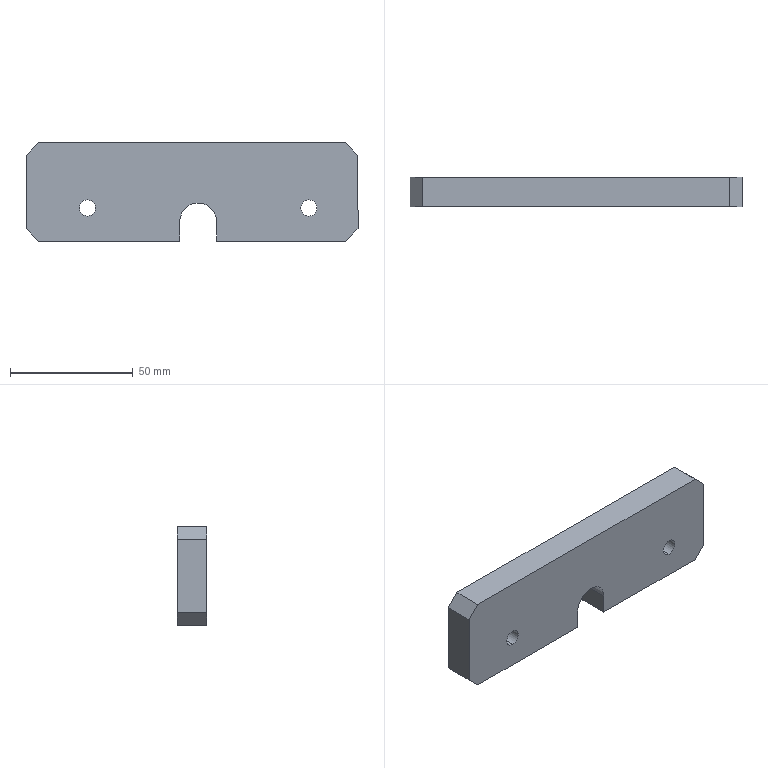Component | SolidWorks | PressingMechanism-26-1 | 1 solid | 18 faces | box 135 x 12 x 40 mm | volume 60879 mm3 | plane 13 | cylinder 5 | commonest cylinder face diameters 6.6 x4 15 x1
build123d program:
from build123d import *

# Parameters (mm, degrees)
SKETCH1_W               = 140
SKETCH1_H               = 50
EXTRUDE1_DEPTH          = 6
M6_CLEARANCE_HOLE1_D    = 6.6
CUT_EXTRUDE1_DEPTH      = 76.293
SKETCH2_W               = 140
SKETCH2_H               = 12.913
CUT_EXTRUDE1_2_DEPTH    = 25
CHAMFER1_SIZE           = 5
CUT_EXTRUDE2_DEPTH      = 76.293
CUT_EXTRUDE2_DEPTH_BACK = 76.293
CHAMFER1_2_SIZE         = 5


with BuildPart() as part:
    # Sketch1 → Extrude1 (new, symmetric)
    with BuildSketch(Plane(origin=(0, 0, 0), x_dir=(1, 0, 0), z_dir=(0, 1, 0))):
        Rectangle(SKETCH1_W, SKETCH1_H)
    extrude(amount=EXTRUDE1_DEPTH, both=True)

    # M6 Clearance Hole1 (through all)
    with Locations(Plane(origin=(0, -6, 0), x_dir=(-1, 0, 0), z_dir=(0, -1, 0))):
        with Locations((45, -1.5), (-45, -1.5)):
            Hole(M6_CLEARANCE_HOLE1_D / 2)

    # Sketch7 → Cut-Extrude1 (cut, through all)
    with BuildSketch(Plane(origin=(0, 6, 0), x_dir=(1, 0, 0), z_dir=(0, 1, 0))):
        with BuildLine():
            Line((7.5, -25), (7.5, -7))
            ThreePointArc((7.5, -7), (0, 0.5), (-7.5, -7))
            Line((-7.5, -7), (-7.5, -25))
            Line((-7.5, -25), (7.5, -25))
        make_face()
    extrude(amount=-CUT_EXTRUDE1_DEPTH, mode=Mode.SUBTRACT)

    # Sketch2 → Cut-Extrude1_2 (cut)
    with BuildSketch(Plane(origin=(0, 6, 0), x_dir=(1, 0, 0), z_dir=(0, 1, 0))):
        with Locations((0, -21.457)):
            Rectangle(SKETCH2_W, SKETCH2_H)
    extrude(amount=-CUT_EXTRUDE1_2_DEPTH, mode=Mode.SUBTRACT)

    # Chamfer1
    chamfer1_edges = [part.edges().sort_by_distance(p)[0] for p in [
        (70, 0, 15),
        (-70, 0, 15),
        (-70, 0, -25),
        (70, 0, -25),
    ]]
    chamfer(chamfer1_edges, length=CHAMFER1_SIZE)

    # Sketch3_2 → Cut-Extrude2 (cut, two sides: drawn at the far end of the back side and taken through both)
    with BuildSketch(Plane.XZ.offset(6).offset(-CUT_EXTRUDE2_DEPTH_BACK)):
        Polygon((65, 307.002), (65, 15), (65, -25.698), (65, -317.7), (649.005, -317.7), (649.005, 307.002), align=None)
    extrude(amount=CUT_EXTRUDE2_DEPTH + CUT_EXTRUDE2_DEPTH_BACK, mode=Mode.SUBTRACT)

    # Chamfer1_2
    chamfer1_2_edges = [part.edges().sort_by_distance(p)[0] for p in [
        (65, 0, 15),
        (65, 0, -25),
    ]]
    chamfer(chamfer1_2_edges, length=CHAMFER1_2_SIZE)


solid = part.part

# Placed as in the assembly
solid = solid.moved(Location((45, -265, 62.5), (180, 0, 0)))
STEP:
#1=COLOUR_RGB('',0.7922,0.8196,0.9333);
#2=FILL_AREA_STYLE_COLOUR('',#1);
#3=FILL_AREA_STYLE('',(#2));
#4=SURFACE_STYLE_FILL_AREA(#3);
#5=SURFACE_SIDE_STYLE('',(#4));
#6=SURFACE_STYLE_USAGE(.BOTH.,#5);
#7=PRESENTATION_STYLE_ASSIGNMENT((#6));
#8=CARTESIAN_POINT('',(-0.,-10.669,2.272));
#9=VERTEX_POINT('',#8);
#10=CARTESIAN_POINT('',(-0.,-10.669,2.531));
#11=VERTEX_POINT('',#10);
#12=CARTESIAN_POINT('',(-0.,-10.669,2.402));
#13=DIRECTION('',(0.,1.,0.));
#14=DIRECTION('',(-0.,0.,1.));
#15=AXIS2_PLACEMENT_3D('',#12,#13,#14);
#16=CIRCLE('',#15,0.1299);
#17=EDGE_CURVE('',#9,#11,#16,.T.);
#18=ORIENTED_EDGE('',*,*,#17,.F.);
#19=CARTESIAN_POINT('',(-0.,-10.197,2.272));
#20=VERTEX_POINT('',#19);
#21=CARTESIAN_POINT('',(-0.,-10.197,2.272));
#22=DIRECTION('',(0.,1.,0.));
#23=VECTOR('',#22,39.37);
#24=LINE('',#21,#23);
#25=EDGE_CURVE('',#9,#20,#24,.T.);
#26=ORIENTED_EDGE('',*,*,#25,.T.);
#27=CARTESIAN_POINT('',(-0.,-10.197,2.531));
#28=VERTEX_POINT('',#27);
#29=CARTESIAN_POINT('',(-0.,-10.197,2.402));
#30=DIRECTION('',(0.,1.,0.));
#31=DIRECTION('',(-0.,0.,1.));
#32=AXIS2_PLACEMENT_3D('',#29,#30,#31);
#33=CIRCLE('',#32,0.1299);
#34=EDGE_CURVE('',#20,#28,#33,.T.);
#35=ORIENTED_EDGE('',*,*,#34,.T.);
#36=CARTESIAN_POINT('',(-0.,-10.197,2.531));
#37=DIRECTION('',(0.,1.,0.));
#38=VECTOR('',#37,39.37);
#39=LINE('',#36,#38);
#40=EDGE_CURVE('',#11,#28,#39,.T.);
#41=ORIENTED_EDGE('',*,*,#40,.F.);
#42=EDGE_LOOP('',(#18,#26,#35,#41));
#43=FACE_OUTER_BOUND('',#42,.T.);
#44=CARTESIAN_POINT('',(-0.,-10.197,2.402));
#45=DIRECTION('',(0.,1.,0.));
#46=DIRECTION('',(-0.,0.,1.));
#47=AXIS2_PLACEMENT_3D('',#44,#45,#46);
#48=CYLINDRICAL_SURFACE('',#47,0.1299);
#49=ADVANCED_FACE('',(#43),#48,.F.);
#50=CARTESIAN_POINT('',(3.543,-10.669,2.272));
#51=VERTEX_POINT('',#50);
#52=CARTESIAN_POINT('',(3.543,-10.669,2.531));
#53=VERTEX_POINT('',#52);
#54=CARTESIAN_POINT('',(3.543,-10.669,2.402));
#55=DIRECTION('',(0.,1.,0.));
#56=DIRECTION('',(0.,0.,1.));
#57=AXIS2_PLACEMENT_3D('',#54,#55,#56);
#58=CIRCLE('',#57,0.1299);
#59=EDGE_CURVE('',#51,#53,#58,.T.);
#60=ORIENTED_EDGE('',*,*,#59,.F.);
#61=CARTESIAN_POINT('',(3.543,-10.197,2.272));
#62=VERTEX_POINT('',#61);
#63=CARTESIAN_POINT('',(3.543,-10.197,2.272));
#64=DIRECTION('',(0.,1.,0.));
#65=VECTOR('',#64,39.37);
#66=LINE('',#63,#65);
#67=EDGE_CURVE('',#51,#62,#66,.T.);
#68=ORIENTED_EDGE('',*,*,#67,.T.);
#69=CARTESIAN_POINT('',(3.543,-10.197,2.531));
#70=VERTEX_POINT('',#69);
#71=CARTESIAN_POINT('',(3.543,-10.197,2.402));
#72=DIRECTION('',(0.,1.,0.));
#73=DIRECTION('',(0.,0.,1.));
#74=AXIS2_PLACEMENT_3D('',#71,#72,#73);
#75=CIRCLE('',#74,0.1299);
#76=EDGE_CURVE('',#62,#70,#75,.T.);
#77=ORIENTED_EDGE('',*,*,#76,.T.);
#78=CARTESIAN_POINT('',(3.543,-10.197,2.531));
#79=DIRECTION('',(0.,1.,0.));
#80=VECTOR('',#79,39.37);
#81=LINE('',#78,#80);
#82=EDGE_CURVE('',#53,#70,#81,.T.);
#83=ORIENTED_EDGE('',*,*,#82,.F.);
#84=EDGE_LOOP('',(#60,#68,#77,#83));
#85=FACE_OUTER_BOUND('',#84,.T.);
#86=CARTESIAN_POINT('',(3.543,-10.197,2.402));
#87=DIRECTION('',(0.,1.,0.));
#88=DIRECTION('',(0.,0.,1.));
#89=AXIS2_PLACEMENT_3D('',#86,#87,#88);
#90=CYLINDRICAL_SURFACE('',#89,0.1299);
#91=ADVANCED_FACE('',(#85),#90,.F.);
#92=CARTESIAN_POINT('',(-0.,-10.669,2.402));
#93=DIRECTION('',(0.,1.,0.));
#94=DIRECTION('',(-0.,0.,1.));
#95=AXIS2_PLACEMENT_3D('',#92,#93,#94);
#96=CIRCLE('',#95,0.1299);
#97=EDGE_CURVE('',#11,#9,#96,.T.);
#98=ORIENTED_EDGE('',*,*,#97,.T.);
#99=ORIENTED_EDGE('',*,*,#17,.T.);
#100=EDGE_LOOP('',(#98,#99));
#101=FACE_BOUND('',#100,.T.);
#102=CARTESIAN_POINT('',(3.543,-10.669,2.402));
#103=DIRECTION('',(0.,1.,0.));
#104=DIRECTION('',(0.,0.,1.));
#105=AXIS2_PLACEMENT_3D('',#102,#103,#104);
#106=CIRCLE('',#105,0.1299);
#107=EDGE_CURVE('',#53,#51,#106,.T.);
#108=ORIENTED_EDGE('',*,*,#107,.T.);
#109=ORIENTED_EDGE('',*,*,#59,.T.);
#110=EDGE_LOOP('',(#108,#109));
#111=FACE_BOUND('',#110,.T.);
#112=CARTESIAN_POINT('',(4.331,-10.669,2.067));
#113=VERTEX_POINT('',#112);
#114=CARTESIAN_POINT('',(4.331,-10.669,3.248));
#115=VERTEX_POINT('',#114);
#116=CARTESIAN_POINT('',(4.331,-10.669,2.461));
#117=DIRECTION('',(-0.,-0.,1.));
#118=VECTOR('',#117,39.37);
#119=LINE('',#116,#118);
#120=EDGE_CURVE('',#113,#115,#119,.T.);
#121=ORIENTED_EDGE('',*,*,#120,.T.);
#122=CARTESIAN_POINT('',(4.134,-10.669,3.445));
#123=VERTEX_POINT('',#122);
#124=CARTESIAN_POINT('',(3.445,-10.669,4.134));
#125=DIRECTION('',(-0.7071,-0.,0.7071));
#126=VECTOR('',#125,39.37);
#127=LINE('',#124,#126);
#128=EDGE_CURVE('',#115,#123,#127,.T.);
#129=ORIENTED_EDGE('',*,*,#128,.T.);
#130=CARTESIAN_POINT('',(-0.7874,-10.669,3.445));
#131=VERTEX_POINT('',#130);
#132=CARTESIAN_POINT('',(-0.9843,-10.669,3.445));
#133=DIRECTION('',(-1.,0.,-0.));
#134=VECTOR('',#133,39.37);
#135=LINE('',#132,#134);
#136=EDGE_CURVE('',#123,#131,#135,.T.);
#137=ORIENTED_EDGE('',*,*,#136,.T.);
#138=CARTESIAN_POINT('',(-0.9843,-10.669,3.248));
#139=VERTEX_POINT('',#138);
#140=CARTESIAN_POINT('',(0.,-10.669,4.232));
#141=DIRECTION('',(-0.7071,0.,-0.7071));
#142=VECTOR('',#141,39.37);
#143=LINE('',#140,#142);
#144=EDGE_CURVE('',#131,#139,#143,.T.);
#145=ORIENTED_EDGE('',*,*,#144,.T.);
#146=CARTESIAN_POINT('',(-0.9843,-10.669,2.067));
#147=VERTEX_POINT('',#146);
#148=CARTESIAN_POINT('',(-0.9843,-10.669,3.445));
#149=DIRECTION('',(0.,0.,-1.));
#150=VECTOR('',#149,39.37);
#151=LINE('',#148,#150);
#152=EDGE_CURVE('',#139,#147,#151,.T.);
#153=ORIENTED_EDGE('',*,*,#152,.T.);
#154=CARTESIAN_POINT('',(-0.7874,-10.669,1.87));
#155=VERTEX_POINT('',#154);
#156=CARTESIAN_POINT('',(0.1969,-10.669,0.8858));
#157=DIRECTION('',(0.7071,0.,-0.7071));
#158=VECTOR('',#157,39.37);
#159=LINE('',#156,#158);
#160=EDGE_CURVE('',#147,#155,#159,.T.);
#161=ORIENTED_EDGE('',*,*,#160,.T.);
#162=CARTESIAN_POINT('',(1.476,-10.669,1.87));
#163=VERTEX_POINT('',#162);
#164=CARTESIAN_POINT('',(-0.9843,-10.669,1.87));
#165=DIRECTION('',(-1.,0.,-0.));
#166=VECTOR('',#165,39.37);
#167=LINE('',#164,#166);
#168=EDGE_CURVE('',#163,#155,#167,.T.);
#169=ORIENTED_EDGE('',*,*,#168,.F.);
#170=CARTESIAN_POINT('',(1.476,-10.669,2.185));
#171=VERTEX_POINT('',#170);
#172=CARTESIAN_POINT('',(1.476,-10.669,1.476));
#173=DIRECTION('',(-0.,0.,-1.));
#174=VECTOR('',#173,39.37);
#175=LINE('',#172,#174);
#176=EDGE_CURVE('',#171,#163,#175,.T.);
#177=ORIENTED_EDGE('',*,*,#176,.F.);
#178=CARTESIAN_POINT('',(2.067,-10.669,2.185));
#179=VERTEX_POINT('',#178);
#180=CARTESIAN_POINT('',(1.772,-10.669,2.185));
#181=DIRECTION('',(-0.,-1.,-0.));
#182=DIRECTION('',(0.,0.,1.));
#183=AXIS2_PLACEMENT_3D('',#180,#181,#182);
#184=CIRCLE('',#183,0.2953);
#185=EDGE_CURVE('',#179,#171,#184,.T.);
#186=ORIENTED_EDGE('',*,*,#185,.F.);
#187=CARTESIAN_POINT('',(2.067,-10.669,1.87));
#188=VERTEX_POINT('',#187);
#189=CARTESIAN_POINT('',(2.067,-10.669,1.476));
#190=DIRECTION('',(-0.,-0.,1.));
#191=VECTOR('',#190,39.37);
#192=LINE('',#189,#191);
#193=EDGE_CURVE('',#188,#179,#192,.T.);
#194=ORIENTED_EDGE('',*,*,#193,.F.);
#195=CARTESIAN_POINT('',(4.134,-10.669,1.87));
#196=VERTEX_POINT('',#195);
#197=CARTESIAN_POINT('',(-0.9843,-10.669,1.87));
#198=DIRECTION('',(-1.,0.,-0.));
#199=VECTOR('',#198,39.37);
#200=LINE('',#197,#199);
#201=EDGE_CURVE('',#196,#188,#200,.T.);
#202=ORIENTED_EDGE('',*,*,#201,.F.);
#203=CARTESIAN_POINT('',(3.248,-10.669,0.9843));
#204=DIRECTION('',(0.7071,-0.,0.7071));
#205=VECTOR('',#204,39.37);
#206=LINE('',#203,#205);
#207=EDGE_CURVE('',#196,#113,#206,.T.);
#208=ORIENTED_EDGE('',*,*,#207,.T.);
#209=EDGE_LOOP('',(#121,#129,#137,#145,#153,#161,#169,#177,#186,#194,#202,#208));
#210=FACE_OUTER_BOUND('',#209,.T.);
#211=CARTESIAN_POINT('',(1.772,-10.669,2.461));
#212=DIRECTION('',(-0.,-1.,-0.));
#213=DIRECTION('',(0.,0.,-1.));
#214=AXIS2_PLACEMENT_3D('',#211,#212,#213);
#215=PLANE('',#214);
#216=ADVANCED_FACE('',(#101,#111,#210),#215,.T.);
#217=CARTESIAN_POINT('',(3.543,-10.197,2.402));
#218=DIRECTION('',(0.,1.,0.));
#219=DIRECTION('',(0.,0.,1.));
#220=AXIS2_PLACEMENT_3D('',#217,#218,#219);
#221=CIRCLE('',#220,0.1299);
#222=EDGE_CURVE('',#70,#62,#221,.T.);
#223=ORIENTED_EDGE('',*,*,#222,.F.);
#224=ORIENTED_EDGE('',*,*,#76,.F.);
#225=EDGE_LOOP('',(#223,#224));
#226=FACE_BOUND('',#225,.T.);
#227=CARTESIAN_POINT('',(-0.,-10.197,2.402));
#228=DIRECTION('',(0.,1.,0.));
#229=DIRECTION('',(-0.,0.,1.));
#230=AXIS2_PLACEMENT_3D('',#227,#228,#229);
#231=CIRCLE('',#230,0.1299);
#232=EDGE_CURVE('',#28,#20,#231,.T.);
#233=ORIENTED_EDGE('',*,*,#232,.F.);
#234=ORIENTED_EDGE('',*,*,#34,.F.);
#235=EDGE_LOOP('',(#233,#234));
#236=FACE_BOUND('',#235,.T.);
#237=CARTESIAN_POINT('',(4.134,-10.197,3.445));
#238=VERTEX_POINT('',#237);
#239=CARTESIAN_POINT('',(-0.7874,-10.197,3.445));
#240=VERTEX_POINT('',#239);
#241=CARTESIAN_POINT('',(-0.9843,-10.197,3.445));
#242=DIRECTION('',(-1.,0.,-0.));
#243=VECTOR('',#242,39.37);
#244=LINE('',#241,#243);
#245=EDGE_CURVE('',#238,#240,#244,.T.);
#246=ORIENTED_EDGE('',*,*,#245,.F.);
#247=CARTESIAN_POINT('',(4.331,-10.197,3.248));
#248=VERTEX_POINT('',#247);
#249=CARTESIAN_POINT('',(4.134,-10.197,3.445));
#250=DIRECTION('',(0.7071,0.,-0.7071));
#251=VECTOR('',#250,39.37);
#252=LINE('',#249,#251);
#253=EDGE_CURVE('',#238,#248,#252,.T.);
#254=ORIENTED_EDGE('',*,*,#253,.T.);
#255=CARTESIAN_POINT('',(4.331,-10.197,2.067));
#256=VERTEX_POINT('',#255);
#257=CARTESIAN_POINT('',(4.331,-10.197,2.461));
#258=DIRECTION('',(-0.,-0.,1.));
#259=VECTOR('',#258,39.37);
#260=LINE('',#257,#259);
#261=EDGE_CURVE('',#256,#248,#260,.T.);
#262=ORIENTED_EDGE('',*,*,#261,.F.);
#263=CARTESIAN_POINT('',(4.134,-10.197,1.87));
#264=VERTEX_POINT('',#263);
#265=CARTESIAN_POINT('',(4.134,-10.197,1.87));
#266=DIRECTION('',(-0.7071,0.,-0.7071));
#267=VECTOR('',#266,39.37);
#268=LINE('',#265,#267);
#269=EDGE_CURVE('',#256,#264,#268,.T.);
#270=ORIENTED_EDGE('',*,*,#269,.T.);
#271=CARTESIAN_POINT('',(2.067,-10.197,1.87));
#272=VERTEX_POINT('',#271);
#273=CARTESIAN_POINT('',(1.772,-10.197,1.87));
#274=DIRECTION('',(-1.,0.,-0.));
#275=VECTOR('',#274,39.37);
#276=LINE('',#273,#275);
#277=EDGE_CURVE('',#264,#272,#276,.T.);
#278=ORIENTED_EDGE('',*,*,#277,.T.);
#279=CARTESIAN_POINT('',(2.067,-10.197,2.185));
#280=VERTEX_POINT('',#279);
#281=CARTESIAN_POINT('',(2.067,-10.197,1.476));
#282=DIRECTION('',(-0.,-0.,1.));
#283=VECTOR('',#282,39.37);
#284=LINE('',#281,#283);
#285=EDGE_CURVE('',#272,#280,#284,.T.);
#286=ORIENTED_EDGE('',*,*,#285,.T.);
#287=CARTESIAN_POINT('',(1.476,-10.197,2.185));
#288=VERTEX_POINT('',#287);
#289=CARTESIAN_POINT('',(1.772,-10.197,2.185));
#290=DIRECTION('',(-0.,-1.,-0.));
#291=DIRECTION('',(0.,0.,1.));
#292=AXIS2_PLACEMENT_3D('',#289,#290,#291);
#293=CIRCLE('',#292,0.2953);
#294=EDGE_CURVE('',#280,#288,#293,.T.);
#295=ORIENTED_EDGE('',*,*,#294,.T.);
#296=CARTESIAN_POINT('',(1.476,-10.197,1.87));
#297=VERTEX_POINT('',#296);
#298=CARTESIAN_POINT('',(1.476,-10.197,1.476));
#299=DIRECTION('',(-0.,0.,-1.));
#300=VECTOR('',#299,39.37);
#301=LINE('',#298,#300);
#302=EDGE_CURVE('',#288,#297,#301,.T.);
#303=ORIENTED_EDGE('',*,*,#302,.T.);
#304=CARTESIAN_POINT('',(-0.7874,-10.197,1.87));
#305=VERTEX_POINT('',#304);
#306=CARTESIAN_POINT('',(1.772,-10.197,1.87));
#307=DIRECTION('',(-1.,0.,-0.));
#308=VECTOR('',#307,39.37);
#309=LINE('',#306,#308);
#310=EDGE_CURVE('',#297,#305,#309,.T.);
#311=ORIENTED_EDGE('',*,*,#310,.T.);
#312=CARTESIAN_POINT('',(-0.9843,-10.197,2.067));
#313=VERTEX_POINT('',#312);
#314=CARTESIAN_POINT('',(-0.9843,-10.197,2.067));
#315=DIRECTION('',(-0.7071,-0.,0.7071));
#316=VECTOR('',#315,39.37);
#317=LINE('',#314,#316);
#318=EDGE_CURVE('',#305,#313,#317,.T.);
#319=ORIENTED_EDGE('',*,*,#318,.T.);
#320=CARTESIAN_POINT('',(-0.9843,-10.197,3.248));
#321=VERTEX_POINT('',#320);
#322=CARTESIAN_POINT('',(-0.9843,-10.197,3.445));
#323=DIRECTION('',(0.,0.,-1.));
#324=VECTOR('',#323,39.37);
#325=LINE('',#322,#324);
#326=EDGE_CURVE('',#321,#313,#325,.T.);
#327=ORIENTED_EDGE('',*,*,#326,.F.);
#328=CARTESIAN_POINT('',(-0.9843,-10.197,3.248));
#329=DIRECTION('',(0.7071,-0.,0.7071));
#330=VECTOR('',#329,39.37);
#331=LINE('',#328,#330);
#332=EDGE_CURVE('',#321,#240,#331,.T.);
#333=ORIENTED_EDGE('',*,*,#332,.T.);
#334=EDGE_LOOP('',(#246,#254,#262,#270,#278,#286,#295,#303,#311,#319,#327,#333));
#335=FACE_OUTER_BOUND('',#334,.T.);
#336=CARTESIAN_POINT('',(1.772,-10.197,2.461));
#337=DIRECTION('',(-0.,-1.,-0.));
#338=DIRECTION('',(0.,0.,-1.));
#339=AXIS2_PLACEMENT_3D('',#336,#337,#338);
#340=PLANE('',#339);
#341=ADVANCED_FACE('',(#226,#236,#335),#340,.F.);
#342=ORIENTED_EDGE('',*,*,#326,.T.);
#343=CARTESIAN_POINT('',(-0.9843,-10.669,2.067));
#344=DIRECTION('',(-0.,-1.,-0.));
#345=VECTOR('',#344,39.37);
#346=LINE('',#343,#345);
#347=EDGE_CURVE('',#313,#147,#346,.T.);
#348=ORIENTED_EDGE('',*,*,#347,.T.);
#349=ORIENTED_EDGE('',*,*,#152,.F.);
#350=CARTESIAN_POINT('',(-0.9843,-10.669,3.248));
#351=DIRECTION('',(0.,1.,0.));
#352=VECTOR('',#351,39.37);
#353=LINE('',#350,#352);
#354=EDGE_CURVE('',#139,#321,#353,.T.);
#355=ORIENTED_EDGE('',*,*,#354,.T.);
#356=EDGE_LOOP('',(#342,#348,#349,#355));
#357=FACE_OUTER_BOUND('',#356,.T.);
#358=CARTESIAN_POINT('',(-0.9843,-10.669,3.445));
#359=DIRECTION('',(1.,-0.,0.));
#360=DIRECTION('',(-0.,-0.,1.));
#361=AXIS2_PLACEMENT_3D('',#358,#359,#360);
#362=PLANE('',#361);
#363=ADVANCED_FACE('',(#357),#362,.F.);
#364=ORIENTED_EDGE('',*,*,#136,.F.);
#365=CARTESIAN_POINT('',(4.134,-10.197,3.445));
#366=DIRECTION('',(0.,1.,0.));
#367=VECTOR('',#366,39.37);
#368=LINE('',#365,#367);
#369=EDGE_CURVE('',#123,#238,#368,.T.);
#370=ORIENTED_EDGE('',*,*,#369,.T.);
#371=ORIENTED_EDGE('',*,*,#245,.T.);
#372=CARTESIAN_POINT('',(-0.7874,-10.669,3.445));
#373=DIRECTION('',(-0.,-1.,-0.));
#374=VECTOR('',#373,39.37);
#375=LINE('',#372,#374);
#376=EDGE_CURVE('',#240,#131,#375,.T.);
#377=ORIENTED_EDGE('',*,*,#376,.T.);
#378=EDGE_LOOP('',(#364,#370,#371,#377));
#379=FACE_OUTER_BOUND('',#378,.T.);
#380=CARTESIAN_POINT('',(-0.9843,-10.669,3.445));
#381=DIRECTION('',(0.,0.,-1.));
#382=DIRECTION('',(1.,-0.,0.));
#383=AXIS2_PLACEMENT_3D('',#380,#381,#382);
#384=PLANE('',#383);
#385=ADVANCED_FACE('',(#379),#384,.F.);
#386=ORIENTED_EDGE('',*,*,#67,.F.);
#387=ORIENTED_EDGE('',*,*,#107,.F.);
#388=ORIENTED_EDGE('',*,*,#82,.T.);
#389=ORIENTED_EDGE('',*,*,#222,.T.);
#390=EDGE_LOOP('',(#386,#387,#388,#389));
#391=FACE_OUTER_BOUND('',#390,.T.);
#392=CARTESIAN_POINT('',(3.543,-10.197,2.402));
#393=DIRECTION('',(0.,1.,0.));
#394=DIRECTION('',(0.,0.,1.));
#395=AXIS2_PLACEMENT_3D('',#392,#393,#394);
#396=CYLINDRICAL_SURFACE('',#395,0.1299);
#397=ADVANCED_FACE('',(#391),#396,.F.);
#398=ORIENTED_EDGE('',*,*,#25,.F.);
#399=ORIENTED_EDGE('',*,*,#97,.F.);
#400=ORIENTED_EDGE('',*,*,#40,.T.);
#401=ORIENTED_EDGE('',*,*,#232,.T.);
#402=EDGE_LOOP('',(#398,#399,#400,#401));
#403=FACE_OUTER_BOUND('',#402,.T.);
#404=CARTESIAN_POINT('',(-0.,-10.197,2.402));
#405=DIRECTION('',(0.,1.,0.));
#406=DIRECTION('',(-0.,0.,1.));
#407=AXIS2_PLACEMENT_3D('',#404,#405,#406);
#408=CYLINDRICAL_SURFACE('',#407,0.1299);
#409=ADVANCED_FACE('',(#403),#408,.F.);
#410=ORIENTED_EDGE('',*,*,#185,.T.);
#411=CARTESIAN_POINT('',(1.476,-10.197,2.185));
#412=DIRECTION('',(-0.,-1.,-0.));
#413=VECTOR('',#412,39.37);
#414=LINE('',#411,#413);
#415=EDGE_CURVE('',#288,#171,#414,.T.);
#416=ORIENTED_EDGE('',*,*,#415,.F.);
#417=ORIENTED_EDGE('',*,*,#294,.F.);
#418=CARTESIAN_POINT('',(2.067,-10.197,2.185));
#419=DIRECTION('',(-0.,-1.,-0.));
#420=VECTOR('',#419,39.37);
#421=LINE('',#418,#420);
#422=EDGE_CURVE('',#280,#179,#421,.T.);
#423=ORIENTED_EDGE('',*,*,#422,.T.);
#424=EDGE_LOOP('',(#410,#416,#417,#423));
#425=FACE_OUTER_BOUND('',#424,.T.);
#426=CARTESIAN_POINT('',(1.772,-10.197,2.185));
#427=DIRECTION('',(-0.,-1.,-0.));
#428=DIRECTION('',(0.,0.,-1.));
#429=AXIS2_PLACEMENT_3D('',#426,#427,#428);
#430=CYLINDRICAL_SURFACE('',#429,0.2953);
#431=ADVANCED_FACE('',(#425),#430,.F.);
#432=ORIENTED_EDGE('',*,*,#285,.F.);
#433=CARTESIAN_POINT('',(2.067,-10.197,1.87));
#434=DIRECTION('',(-0.,-1.,-0.));
#435=VECTOR('',#434,39.37);
#436=LINE('',#433,#435);
#437=EDGE_CURVE('',#272,#188,#436,.T.);
#438=ORIENTED_EDGE('',*,*,#437,.T.);
#439=ORIENTED_EDGE('',*,*,#193,.T.);
#440=ORIENTED_EDGE('',*,*,#422,.F.);
#441=EDGE_LOOP('',(#432,#438,#439,#440));
#442=FACE_OUTER_BOUND('',#441,.T.);
#443=CARTESIAN_POINT('',(2.067,-10.197,1.476));
#444=DIRECTION('',(1.,-0.,0.));
#445=DIRECTION('',(-0.,-0.,1.));
#446=AXIS2_PLACEMENT_3D('',#443,#444,#445);
#447=PLANE('',#446);
#448=ADVANCED_FACE('',(#442),#447,.F.);
#449=ORIENTED_EDGE('',*,*,#176,.T.);
#450=CARTESIAN_POINT('',(1.476,-10.197,1.87));
#451=DIRECTION('',(0.,1.,0.));
#452=VECTOR('',#451,39.37);
#453=LINE('',#450,#452);
#454=EDGE_CURVE('',#163,#297,#453,.T.);
#455=ORIENTED_EDGE('',*,*,#454,.T.);
#456=ORIENTED_EDGE('',*,*,#302,.F.);
#457=ORIENTED_EDGE('',*,*,#415,.T.);
#458=EDGE_LOOP('',(#449,#455,#456,#457));
#459=FACE_OUTER_BOUND('',#458,.T.);
#460=CARTESIAN_POINT('',(1.476,-10.197,1.476));
#461=DIRECTION('',(-1.,0.,0.));
#462=DIRECTION('',(-0.,0.,-1.));
#463=AXIS2_PLACEMENT_3D('',#460,#461,#462);
#464=PLANE('',#463);
#465=ADVANCED_FACE('',(#459),#464,.F.);
#466=ORIENTED_EDGE('',*,*,#168,.T.);
#467=CARTESIAN_POINT('',(-0.7874,-9.685,1.87));
#468=DIRECTION('',(0.,1.,0.));
#469=VECTOR('',#468,39.37);
#470=LINE('',#467,#469);
#471=EDGE_CURVE('',#155,#305,#470,.T.);
#472=ORIENTED_EDGE('',*,*,#471,.T.);
#473=ORIENTED_EDGE('',*,*,#310,.F.);
#474=ORIENTED_EDGE('',*,*,#454,.F.);
#475=EDGE_LOOP('',(#466,#472,#473,#474));
#476=FACE_OUTER_BOUND('',#475,.T.);
#477=CARTESIAN_POINT('',(-0.9843,-9.685,1.87));
#478=DIRECTION('',(-0.,-0.,1.));
#479=DIRECTION('',(-1.,0.,-0.));
#480=AXIS2_PLACEMENT_3D('',#477,#478,#479);
#481=PLANE('',#480);
#482=ADVANCED_FACE('',(#476),#481,.F.);
#483=ORIENTED_EDGE('',*,*,#277,.F.);
#484=CARTESIAN_POINT('',(4.134,-10.669,1.87));
#485=DIRECTION('',(-0.,-1.,-0.));
#486=VECTOR('',#485,39.37);
#487=LINE('',#484,#486);
#488=EDGE_CURVE('',#264,#196,#487,.T.);
#489=ORIENTED_EDGE('',*,*,#488,.T.);
#490=ORIENTED_EDGE('',*,*,#201,.T.);
#491=ORIENTED_EDGE('',*,*,#437,.F.);
#492=EDGE_LOOP('',(#483,#489,#490,#491));
#493=FACE_OUTER_BOUND('',#492,.T.);
#494=CARTESIAN_POINT('',(-0.9843,-9.685,1.87));
#495=DIRECTION('',(-0.,-0.,1.));
#496=DIRECTION('',(-1.,0.,-0.));
#497=AXIS2_PLACEMENT_3D('',#494,#495,#496);
#498=PLANE('',#497);
#499=ADVANCED_FACE('',(#493),#498,.F.);
#500=ORIENTED_EDGE('',*,*,#318,.F.);
#501=ORIENTED_EDGE('',*,*,#471,.F.);
#502=ORIENTED_EDGE('',*,*,#160,.F.);
#503=ORIENTED_EDGE('',*,*,#347,.F.);
#504=EDGE_LOOP('',(#500,#501,#502,#503));
#505=FACE_OUTER_BOUND('',#504,.T.);
#506=CARTESIAN_POINT('',(-0.9843,-10.669,2.067));
#507=DIRECTION('',(0.7071,-0.,0.7071));
#508=DIRECTION('',(-0.,-1.,-0.));
#509=AXIS2_PLACEMENT_3D('',#506,#507,#508);
#510=PLANE('',#509);
#511=ADVANCED_FACE('',(#505),#510,.F.);
#512=ORIENTED_EDGE('',*,*,#144,.F.);
#513=ORIENTED_EDGE('',*,*,#376,.F.);
#514=ORIENTED_EDGE('',*,*,#332,.F.);
#515=ORIENTED_EDGE('',*,*,#354,.F.);
#516=EDGE_LOOP('',(#512,#513,#514,#515));
#517=FACE_OUTER_BOUND('',#516,.T.);
#518=CARTESIAN_POINT('',(-0.9843,-10.669,3.248));
#519=DIRECTION('',(0.7071,0.,-0.7071));
#520=DIRECTION('',(0.,1.,0.));
#521=AXIS2_PLACEMENT_3D('',#518,#519,#520);
#522=PLANE('',#521);
#523=ADVANCED_FACE('',(#517),#522,.F.);
#524=ORIENTED_EDGE('',*,*,#261,.T.);
#525=CARTESIAN_POINT('',(4.331,-10.669,3.248));
#526=DIRECTION('',(-0.,-1.,-0.));
#527=VECTOR('',#526,39.37);
#528=LINE('',#525,#527);
#529=EDGE_CURVE('',#248,#115,#528,.T.);
#530=ORIENTED_EDGE('',*,*,#529,.T.);
#531=ORIENTED_EDGE('',*,*,#120,.F.);
#532=CARTESIAN_POINT('',(4.331,-10.197,2.067));
#533=DIRECTION('',(0.,1.,0.));
#534=VECTOR('',#533,39.37);
#535=LINE('',#532,#534);
#536=EDGE_CURVE('',#113,#256,#535,.T.);
#537=ORIENTED_EDGE('',*,*,#536,.T.);
#538=EDGE_LOOP('',(#524,#530,#531,#537));
#539=FACE_OUTER_BOUND('',#538,.T.);
#540=CARTESIAN_POINT('',(4.331,-3.007,1.87));
#541=DIRECTION('',(1.,-0.,0.));
#542=DIRECTION('',(-0.,-0.,1.));
#543=AXIS2_PLACEMENT_3D('',#540,#541,#542);
#544=PLANE('',#543);
#545=ADVANCED_FACE('',(#539),#544,.T.);
#546=ORIENTED_EDGE('',*,*,#128,.F.);
#547=ORIENTED_EDGE('',*,*,#529,.F.);
#548=ORIENTED_EDGE('',*,*,#253,.F.);
#549=ORIENTED_EDGE('',*,*,#369,.F.);
#550=EDGE_LOOP('',(#546,#547,#548,#549));
#551=FACE_OUTER_BOUND('',#550,.T.);
#552=CARTESIAN_POINT('',(4.134,-10.669,3.445));
#553=DIRECTION('',(0.7071,-0.,0.7071));
#554=DIRECTION('',(-0.,-1.,-0.));
#555=AXIS2_PLACEMENT_3D('',#552,#553,#554);
#556=PLANE('',#555);
#557=ADVANCED_FACE('',(#551),#556,.T.);
#558=ORIENTED_EDGE('',*,*,#269,.F.);
#559=ORIENTED_EDGE('',*,*,#536,.F.);
#560=ORIENTED_EDGE('',*,*,#207,.F.);
#561=ORIENTED_EDGE('',*,*,#488,.F.);
#562=EDGE_LOOP('',(#558,#559,#560,#561));
#563=FACE_OUTER_BOUND('',#562,.T.);
#564=CARTESIAN_POINT('',(4.134,-9.685,1.87));
#565=DIRECTION('',(0.7071,0.,-0.7071));
#566=DIRECTION('',(0.,1.,0.));
#567=AXIS2_PLACEMENT_3D('',#564,#565,#566);
#568=PLANE('',#567);
#569=ADVANCED_FACE('',(#563),#568,.T.);
#570=CLOSED_SHELL('',(#49,#91,#216,#341,#363,#385,#397,#409,#431,#448,#465,#482,#499,#511,#523,#545,#557,#569));
#571=MANIFOLD_SOLID_BREP('',#570);
#572=STYLED_ITEM('',(#7),#571);
#573=PRESENTATION_LAYER_ASSIGNMENT('','',(#572));
#574=CARTESIAN_POINT('',(0.,0.,0.));
#575=DIRECTION('',(0.,0.,1.));
#576=DIRECTION('',(1.,0.,0.));
#577=AXIS2_PLACEMENT_3D('',#574,#575,#576);
#578=(LENGTH_UNIT()NAMED_UNIT(*)SI_UNIT($,.METRE.));
#579=LENGTH_MEASURE_WITH_UNIT(LENGTH_MEASURE(0.0254),#578);
#580=DIMENSIONAL_EXPONENTS(1.,0.,0.,0.,0.,0.,0.);
#581=(CONVERSION_BASED_UNIT('',#579)LENGTH_UNIT()NAMED_UNIT(#580));
#582=UNCERTAINTY_MEASURE_WITH_UNIT(LENGTH_MEASURE(0.00001),#581,'','');
#583=(NAMED_UNIT(*)PLANE_ANGLE_UNIT()SI_UNIT($,.RADIAN.));
#584=(NAMED_UNIT(*)SI_UNIT($,.STERADIAN.)SOLID_ANGLE_UNIT());
#585=(GEOMETRIC_REPRESENTATION_CONTEXT(3)GLOBAL_UNCERTAINTY_ASSIGNED_CONTEXT((#582))GLOBAL_UNIT_ASSIGNED_CONTEXT((#581,#583,#584))REPRESENTATION_CONTEXT('',''));
#586=ADVANCED_BREP_SHAPE_REPRESENTATION('',(#571,#577),#585);
#587=(LENGTH_UNIT()NAMED_UNIT(*)SI_UNIT($,.METRE.));
#588=LENGTH_MEASURE_WITH_UNIT(LENGTH_MEASURE(0.0254),#587);
#589=DIMENSIONAL_EXPONENTS(1.,0.,0.,0.,0.,0.,0.);
#590=(CONVERSION_BASED_UNIT('',#588)LENGTH_UNIT()NAMED_UNIT(#589));
#591=UNCERTAINTY_MEASURE_WITH_UNIT(LENGTH_MEASURE(0.00001),#590,'','');
#592=(NAMED_UNIT(*)PLANE_ANGLE_UNIT()SI_UNIT($,.RADIAN.));
#593=(NAMED_UNIT(*)SI_UNIT($,.STERADIAN.)SOLID_ANGLE_UNIT());
#594=(GEOMETRIC_REPRESENTATION_CONTEXT(3)GLOBAL_UNCERTAINTY_ASSIGNED_CONTEXT((#591))GLOBAL_UNIT_ASSIGNED_CONTEXT((#590,#592,#593))REPRESENTATION_CONTEXT('',''));
#595=MECHANICAL_DESIGN_GEOMETRIC_PRESENTATION_REPRESENTATION('',(#572),#594);